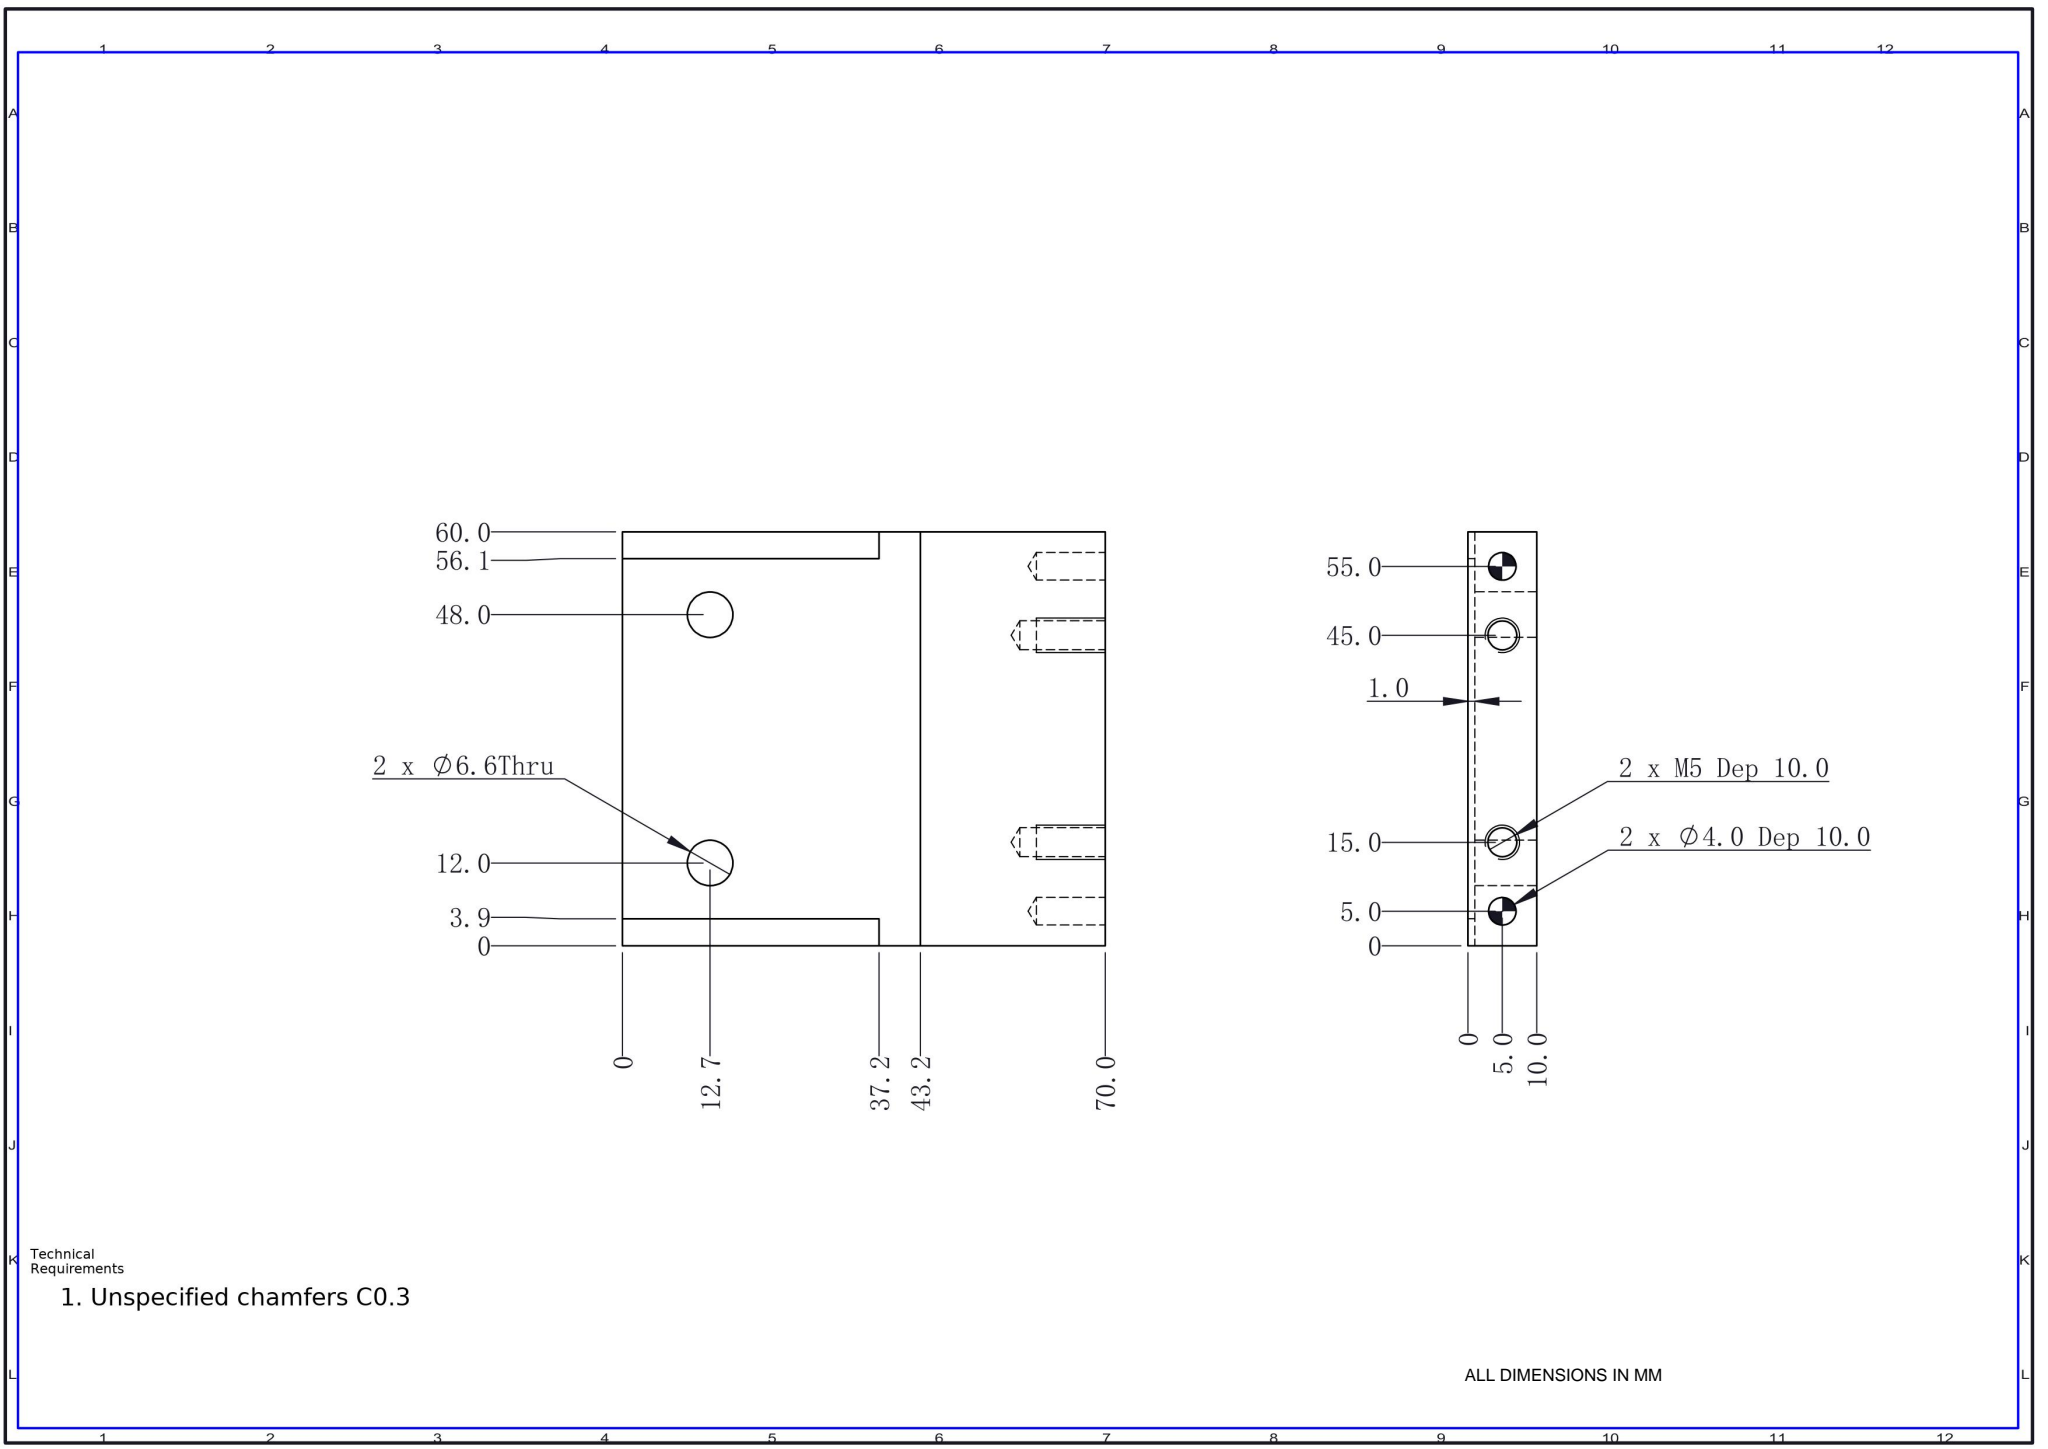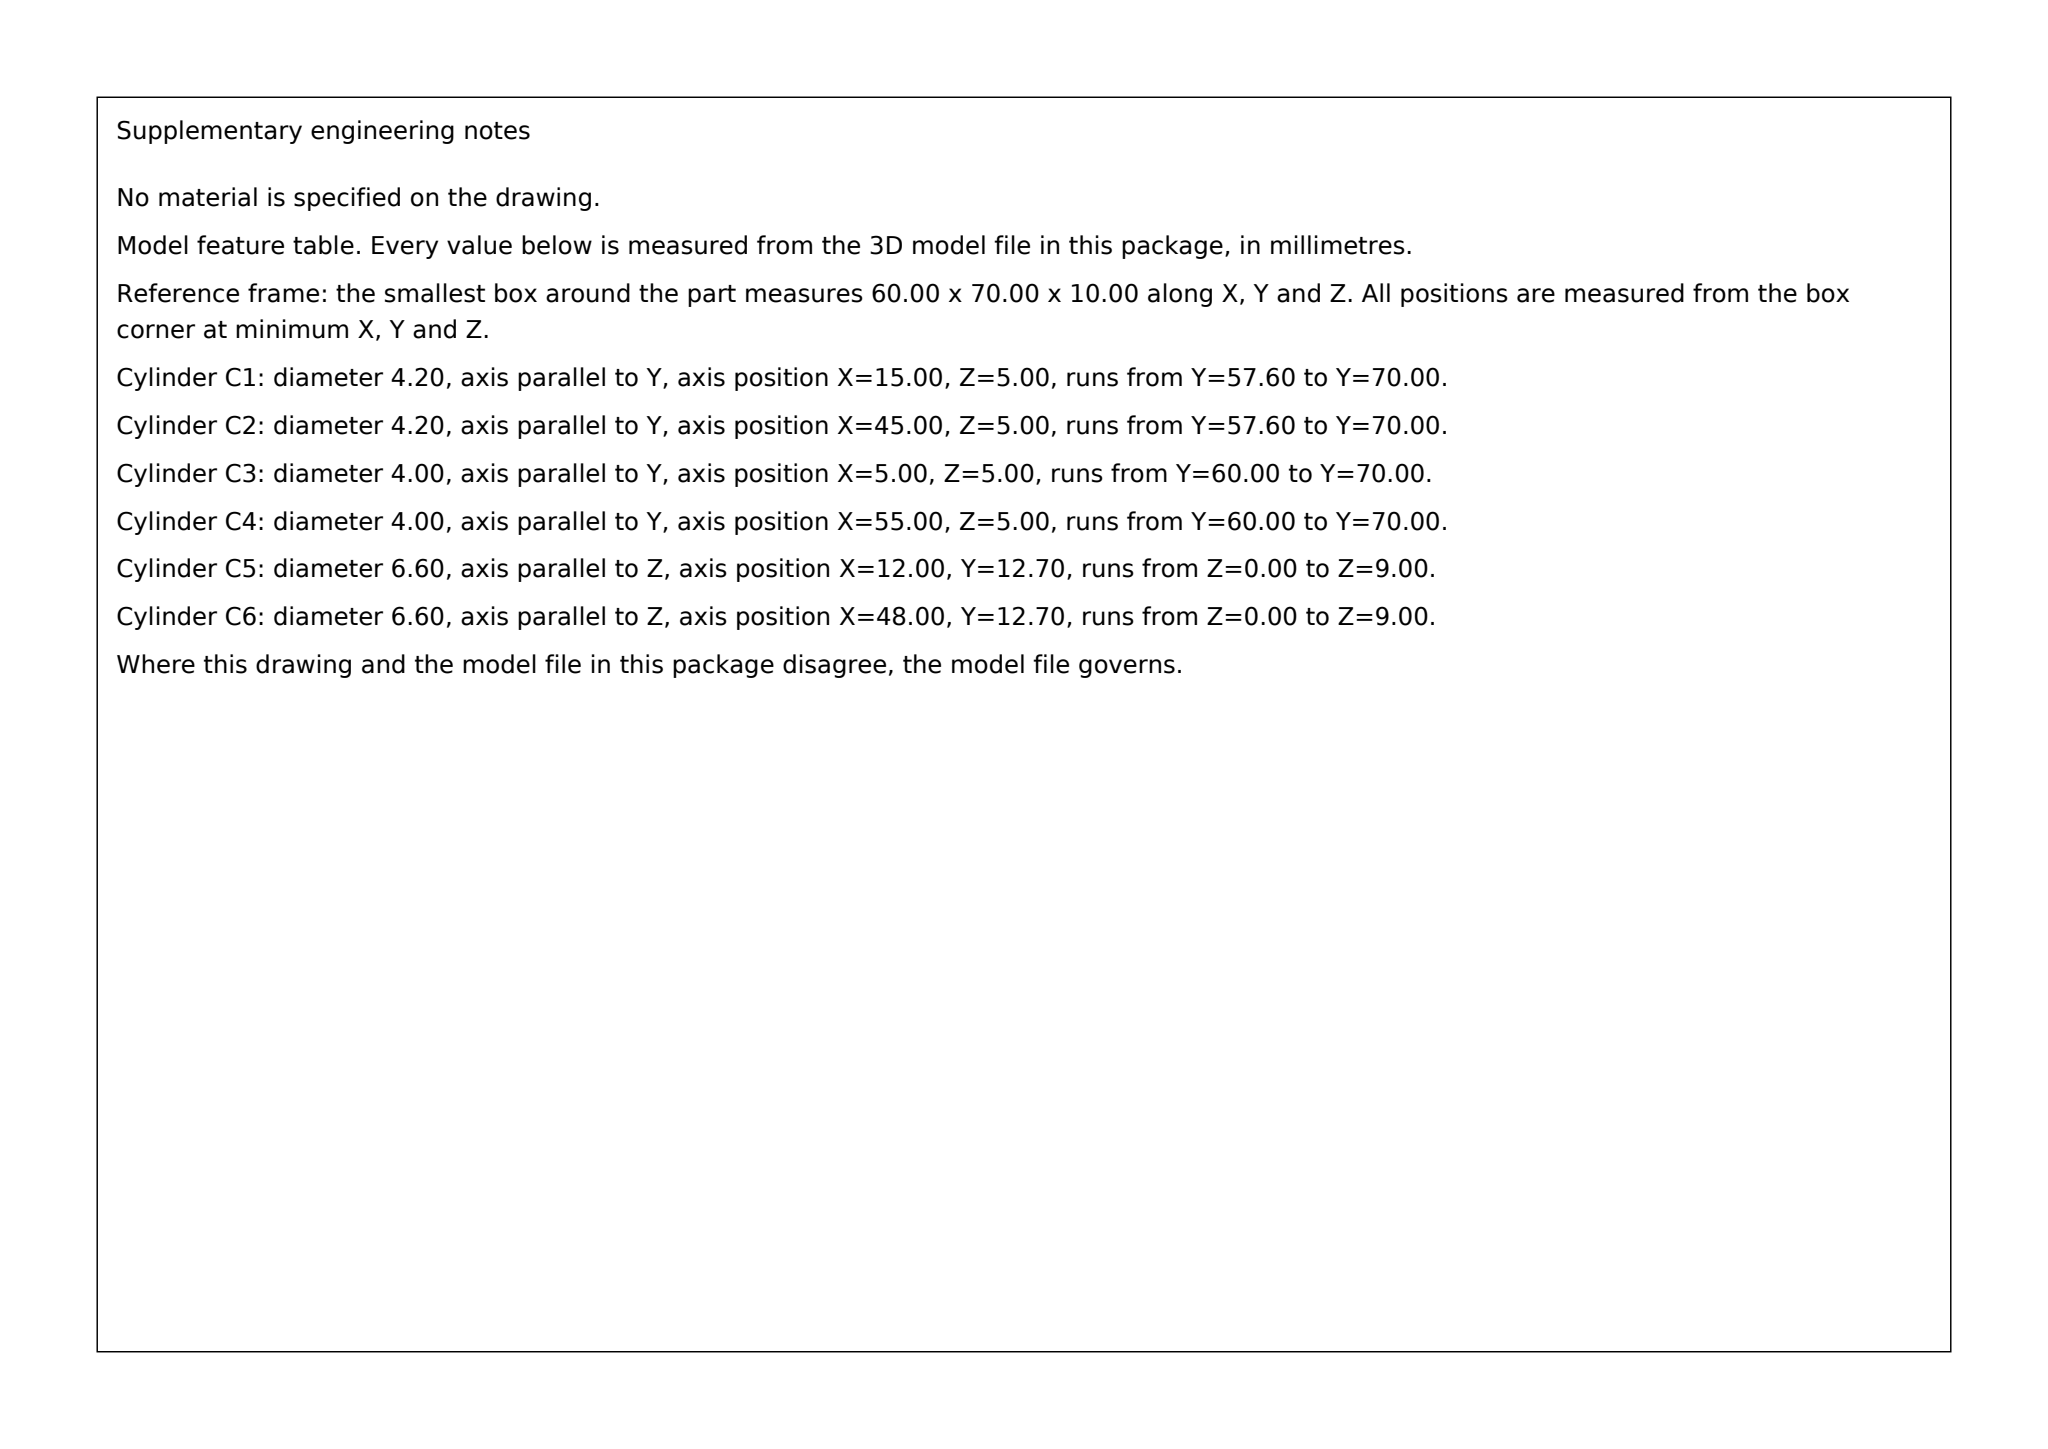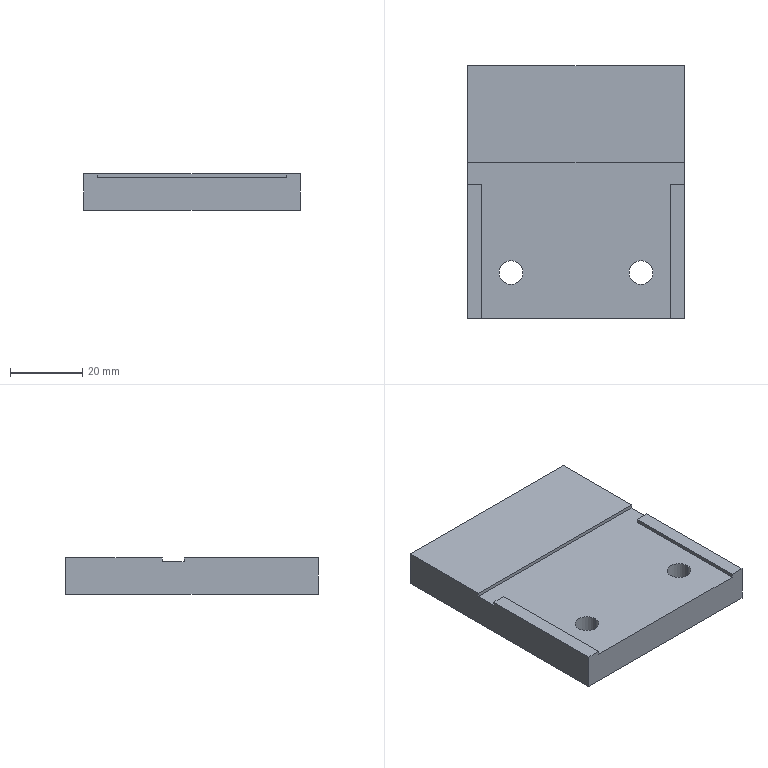Part | SolidWorks | mm | 1 solid | 34 faces | box 60 x 70 x 10 mm | volume 38466 mm3 | plane 14 | cylinder 12 | cone 8 | commonest cylinder face diameters 6.6 x4 4 x4 4.2 x4